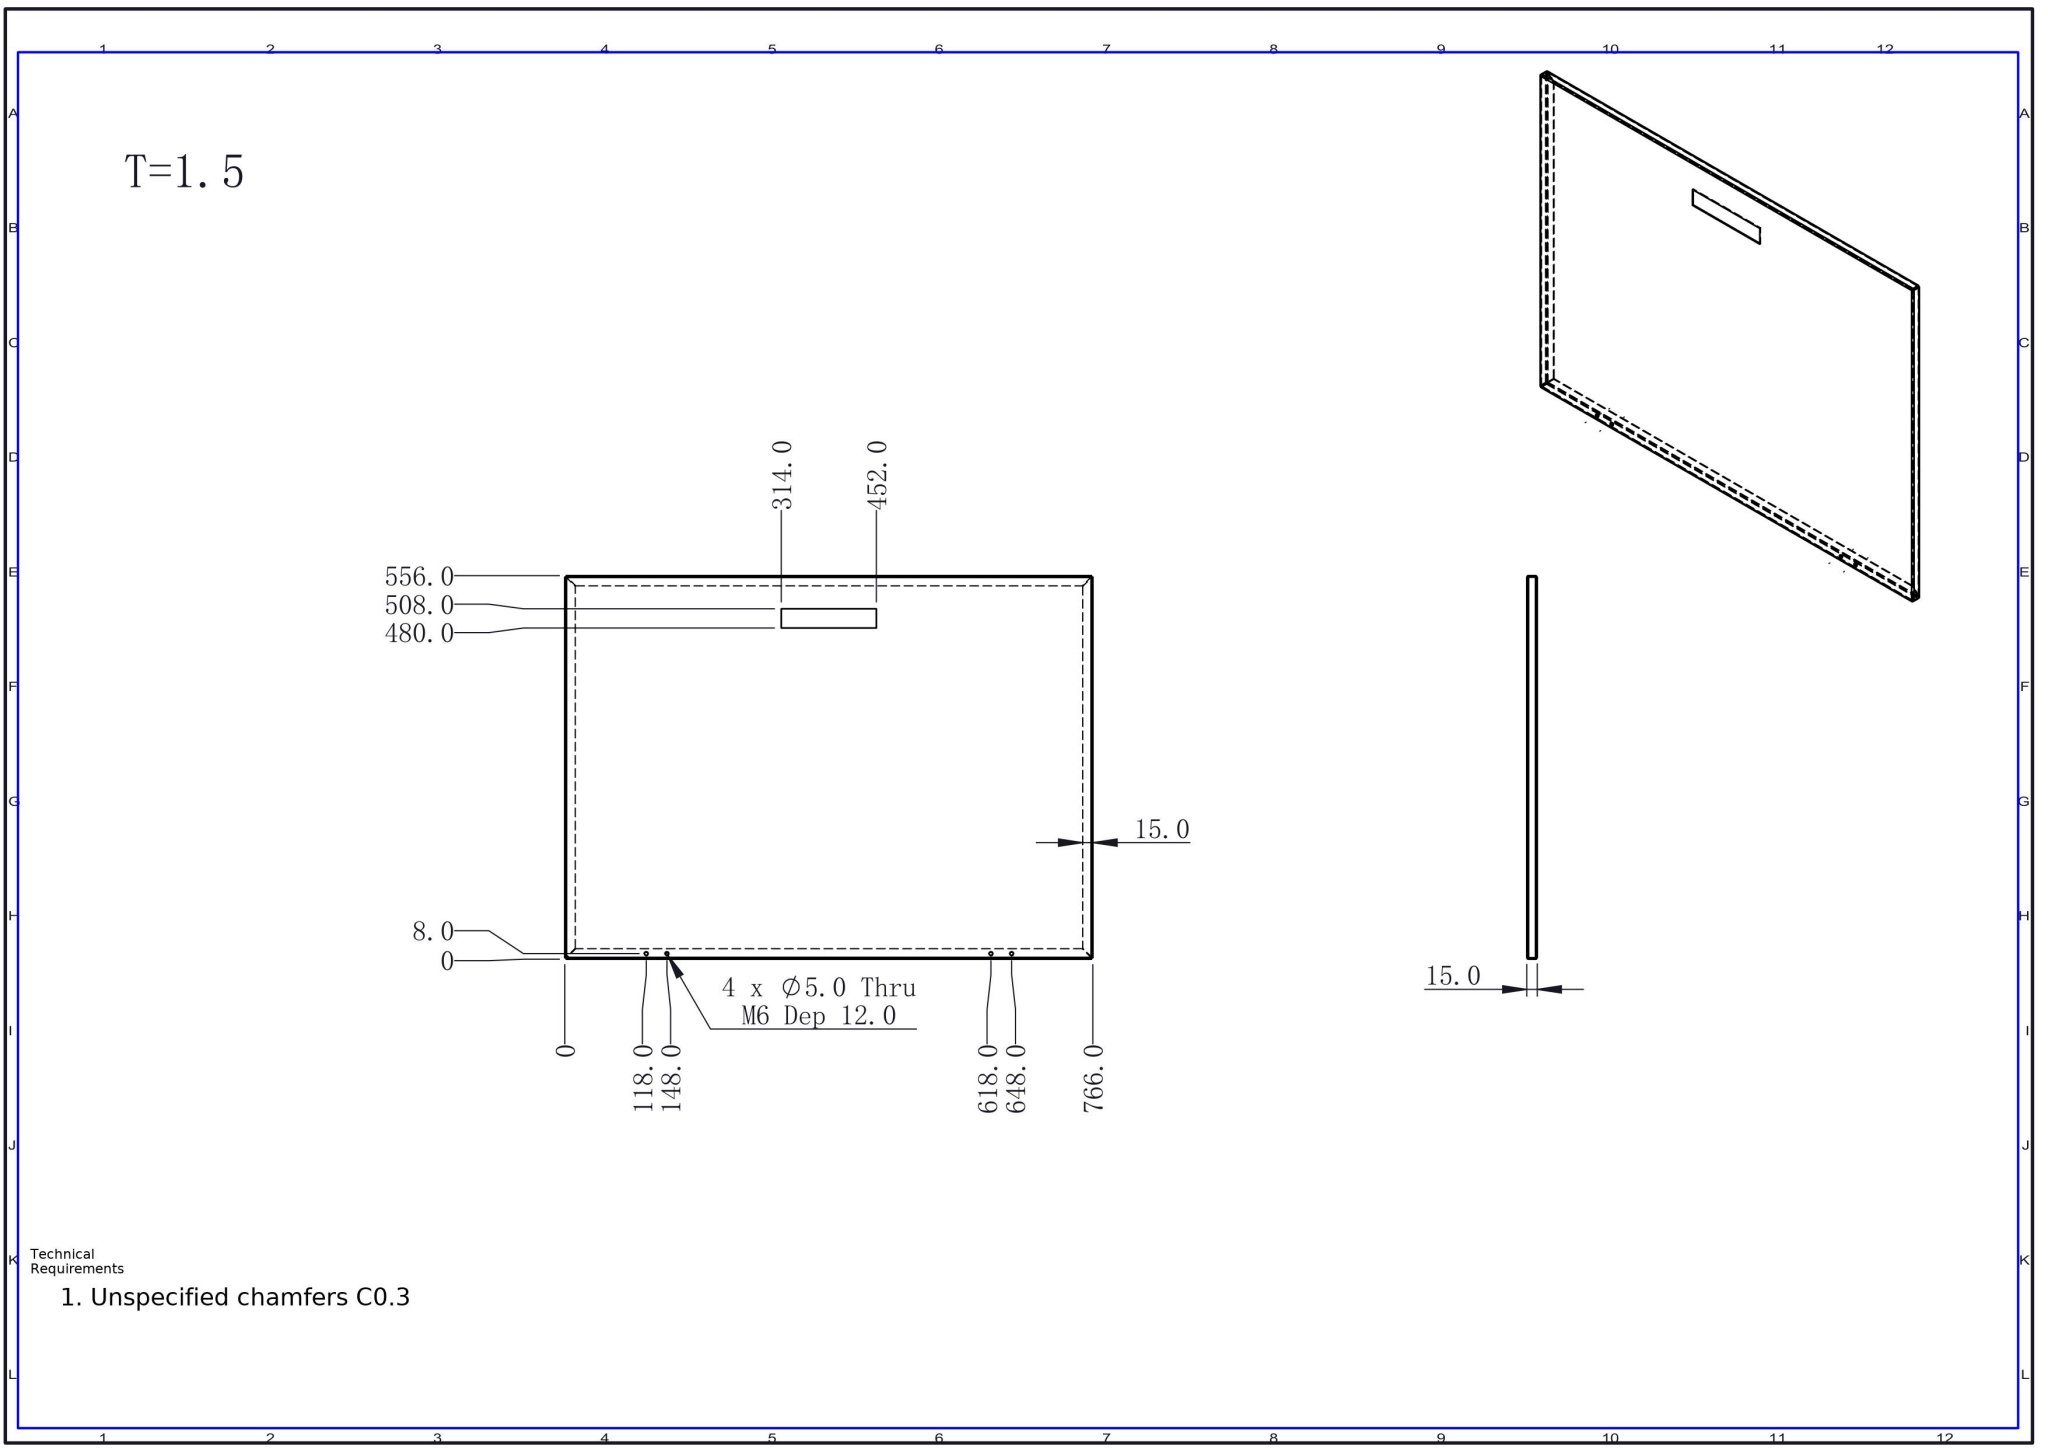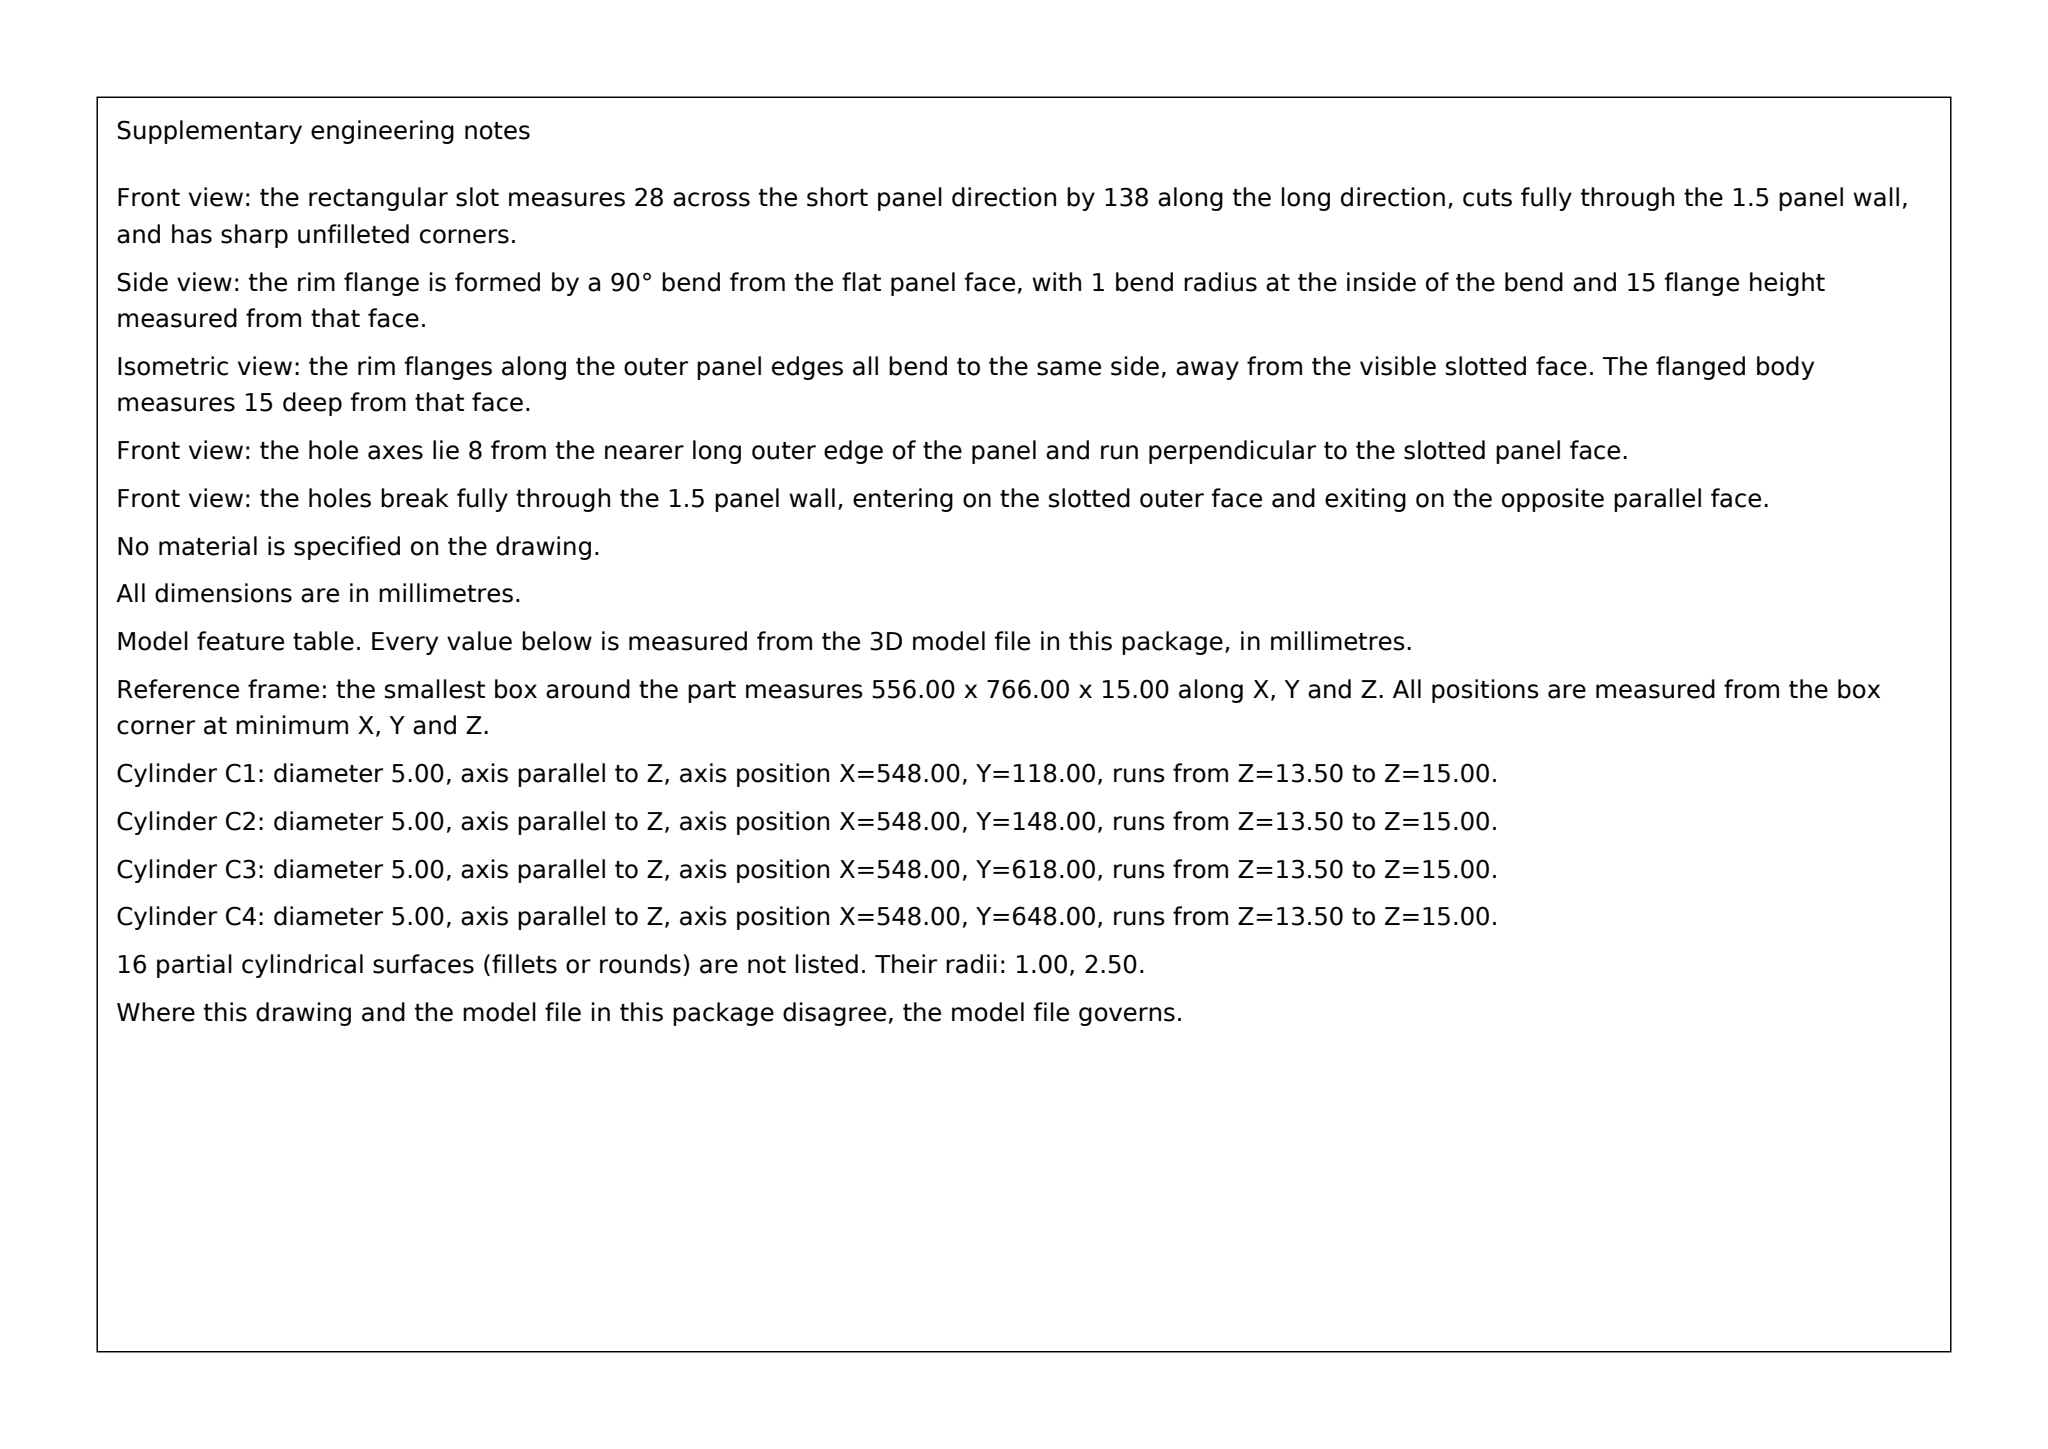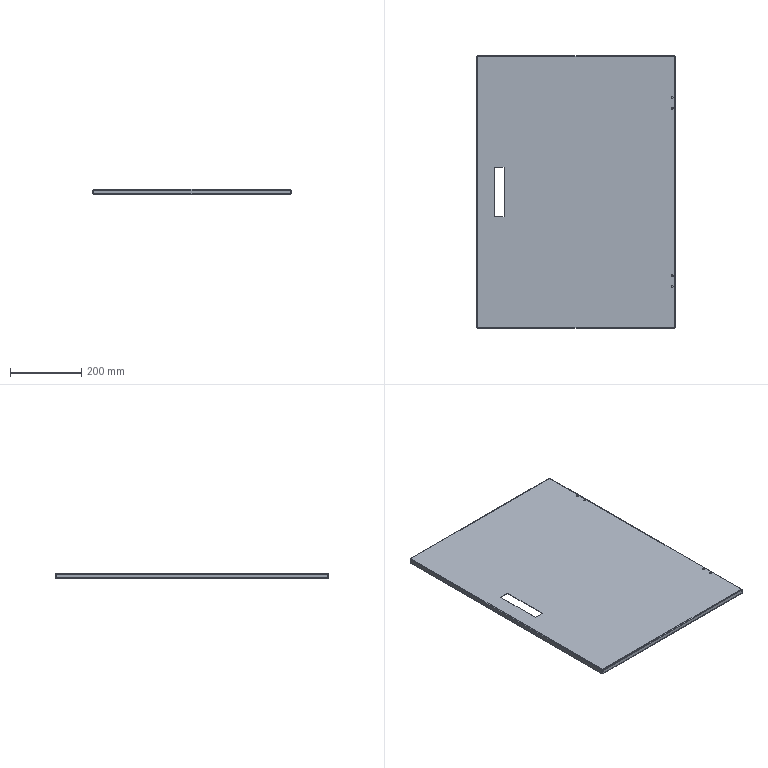Part | SolidWorks | mm | 1 solid | 82 faces | box 556 x 766 x 15 mm | volume 732242 mm3 | plane 42 | cylinder 24 | spline 16 | commonest cylinder face diameters 5 x16 2 x8